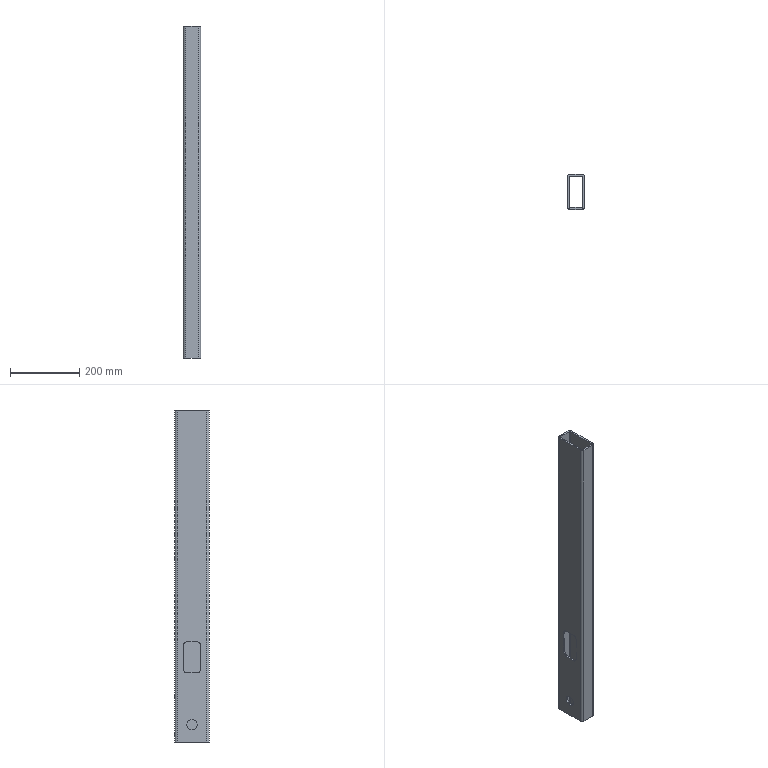Component | SolidWorks | JHK-A1005RightRectangularTubeBeam-1 | 1 solid | 40 faces | box 50 x 100 x 960 mm | volume 1272916 mm3 | cylinder 26 | plane 14 | commonest cylinder face diameters 5 x8 6.8 x6 30 x4 15 x4 20 x4 | material Q235A
build123d program:
from build123d import *

# Parameters (mm, degrees)
EXTRUDE_THIN1_DEPTH   = 480
CUT_EXTRUDE1_REACH    = 487.18
SKETCH2_R             = 15
M8_TAPPED_HOLE1_D     = 6.8
M8_TAPPED_HOLE1_DEPTH = 5
CUT_EXTRUDE2_REACH    = 487.18
CUT_EXTRUDE3_REACH    = 487.18
SKETCH6_R             = 15
M6_TAPPED_HOLE1_D     = 5
M6_TAPPED_HOLE1_DEPTH = 5
M8_TAPPED_HOLE2_D     = 6.8
M8_TAPPED_HOLE2_DEPTH = 5


with BuildPart() as part:
    # Sketch1 → Extrude-Thin1 (new, symmetric)
    with BuildSketch(Plane.XY):
        with BuildLine():
            Line((17.5, 50), (-17.5, 50))
            ThreePointArc((-17.5, 50), (-22.803, 47.803), (-25, 42.5))
            Line((-25, 42.5), (-25, -42.5))
            ThreePointArc((-25, -42.5), (-22.803, -47.803), (-17.5, -50))
            Line((-17.5, -50), (17.5, -50))
            ThreePointArc((17.5, -50), (22.803, -47.803), (25, -42.5))
            Line((25, -42.5), (25, 42.5))
            ThreePointArc((25, 42.5), (22.803, 47.803), (17.5, 50))
        make_face()
        with BuildLine():
            Line((17.5, 45), (-17.5, 45))
            ThreePointArc((-17.5, 45), (-19.268, 44.268), (-20, 42.5))
            Line((-20, 42.5), (-20, -42.5))
            ThreePointArc((-20, -42.5), (-19.268, -44.268), (-17.5, -45))
            Line((-17.5, -45), (17.5, -45))
            ThreePointArc((17.5, -45), (19.268, -44.268), (20, -42.5))
            Line((20, -42.5), (20, 42.5))
            ThreePointArc((20, 42.5), (19.268, 44.268), (17.5, 45))
        make_face(mode=Mode.SUBTRACT)
    extrude(amount=EXTRUDE_THIN1_DEPTH, both=True)

    # Sketch2 → Cut-Extrude1 (cut, up to next)
    with BuildSketch(Plane.ZY.offset(25), mode=Mode.PRIVATE) as cut_extrude1_sk1:
        with Locations((-430, 0)):
            Circle(SKETCH2_R)
    cut_extrude1_tool1 = extrude(cut_extrude1_sk1.sketch, amount=-CUT_EXTRUDE1_REACH, mode=Mode.PRIVATE) & part.part
    add(cut_extrude1_tool1.solids().sort_by_distance((-25, 0, -430))[0], mode=Mode.SUBTRACT)

    # M8 Tapped Hole1
    with Locations(Plane(origin=(25, 29.49, -58.668), x_dir=(0, 0, 1), z_dir=(1, 0, 0))):
        with Locations((338.668, 39.49), (310.668, 39.49)):
            Hole(M8_TAPPED_HOLE1_D / 2, depth=M8_TAPPED_HOLE1_DEPTH)

    # Sketch5 → Cut-Extrude2 (cut, up to next)
    with BuildSketch(Plane(origin=(-25, 0, 0), x_dir=(0, 0, -1), z_dir=(1, 0, 0)), mode=Mode.PRIVATE) as cut_extrude2_sk1:
        with BuildLine():
            Line((200, -25), (270, -25))
            ThreePointArc((270, -25), (277.071, -22.071), (280, -15))
            Line((280, -15), (280, 15))
            ThreePointArc((280, 15), (277.071, 22.071), (270, 25))
            Line((270, 25), (200, 25))
            ThreePointArc((200, 25), (192.929, 22.071), (190, 15))
            Line((190, 15), (190, -15))
            ThreePointArc((190, -15), (192.929, -22.071), (200, -25))
        make_face()
    cut_extrude2_tool1 = extrude(cut_extrude2_sk1.sketch, amount=CUT_EXTRUDE2_REACH, mode=Mode.PRIVATE) & part.part
    add(cut_extrude2_tool1.solids().sort_by_distance((-25, 0, -235))[0], mode=Mode.SUBTRACT)

    # Sketch6 → Cut-Extrude3 (cut, up to next)
    with BuildSketch(Plane(origin=(25, 0, 0), x_dir=(0, 0, -1), z_dir=(1, 0, 0)), mode=Mode.PRIVATE) as cut_extrude3_sk1:
        with Locations((-340, 10)):
            Circle(SKETCH6_R)
    cut_extrude3_tool1 = extrude(cut_extrude3_sk1.sketch, amount=-CUT_EXTRUDE3_REACH, mode=Mode.PRIVATE) & part.part
    add(cut_extrude3_tool1.solids().sort_by_distance((25, 10, 340))[0], mode=Mode.SUBTRACT)

    # M6 Tapped Hole1
    with Locations(Plane(origin=(0, 50, 0), x_dir=(1, 0, 0), z_dir=(0, 1, 0))):
        with Locations((0, 457.5), (0, 347.5)):
            Hole(M6_TAPPED_HOLE1_D / 2, depth=M6_TAPPED_HOLE1_DEPTH)

    # M8 Tapped Hole2
    with Locations(Plane(origin=(0, 50, 0), x_dir=(1, 0, 0), z_dir=(0, 1, 0))):
        with Locations((0, -50)):
            Hole(M8_TAPPED_HOLE2_D / 2, depth=M8_TAPPED_HOLE2_DEPTH)


solid = part.part

# Placed as in the assembly
solid = solid.moved(Location((155, -105, -761), (0, 0, 0)))